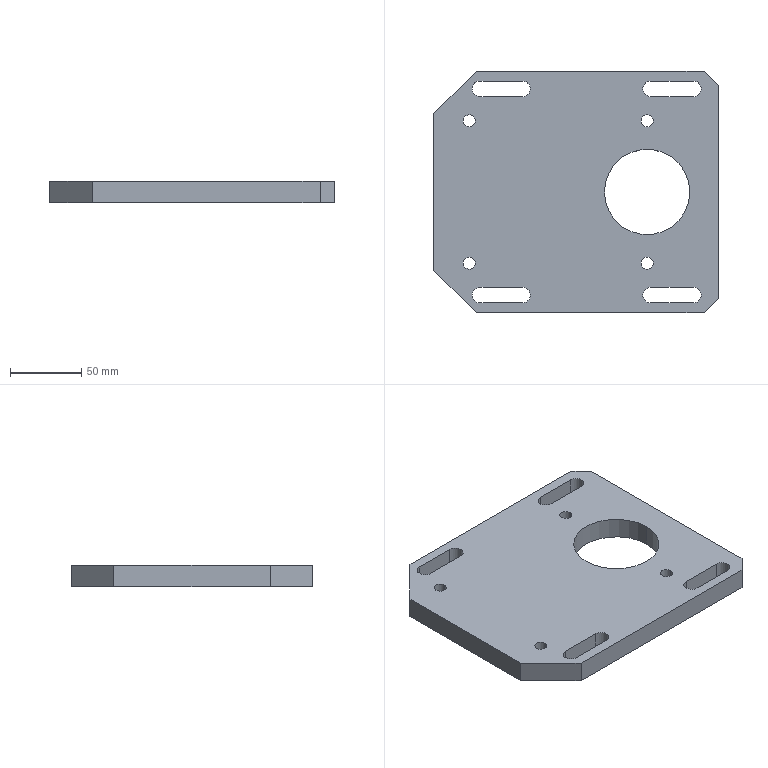CAM job | Mastercam | mm | 8 operations | part box 200 x 170 x 15
1. Contour (Ramp) | 1 - 8 平铣刀
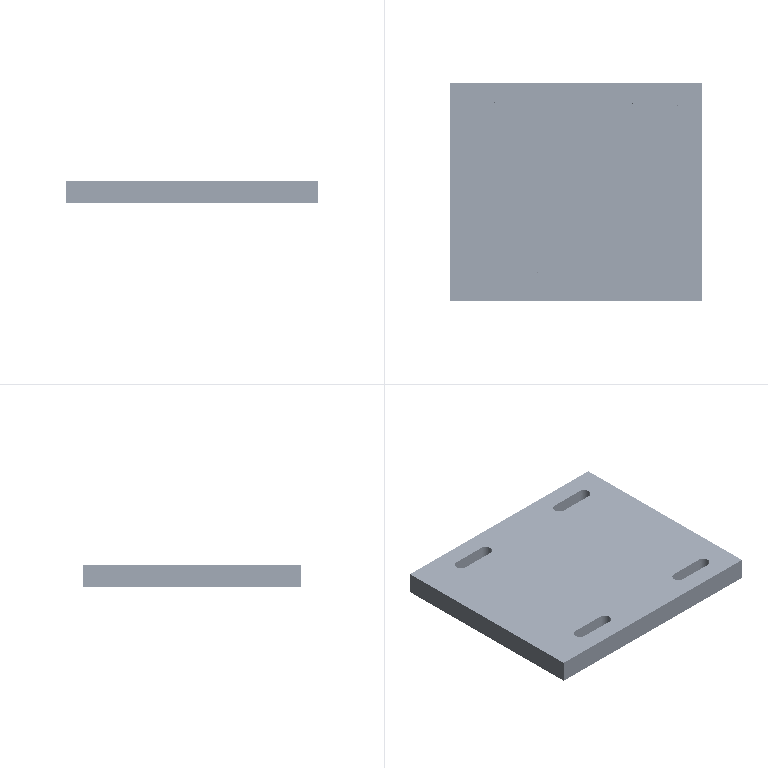2. 3D High Speed (Waterline) | 1 - 8 平铣刀
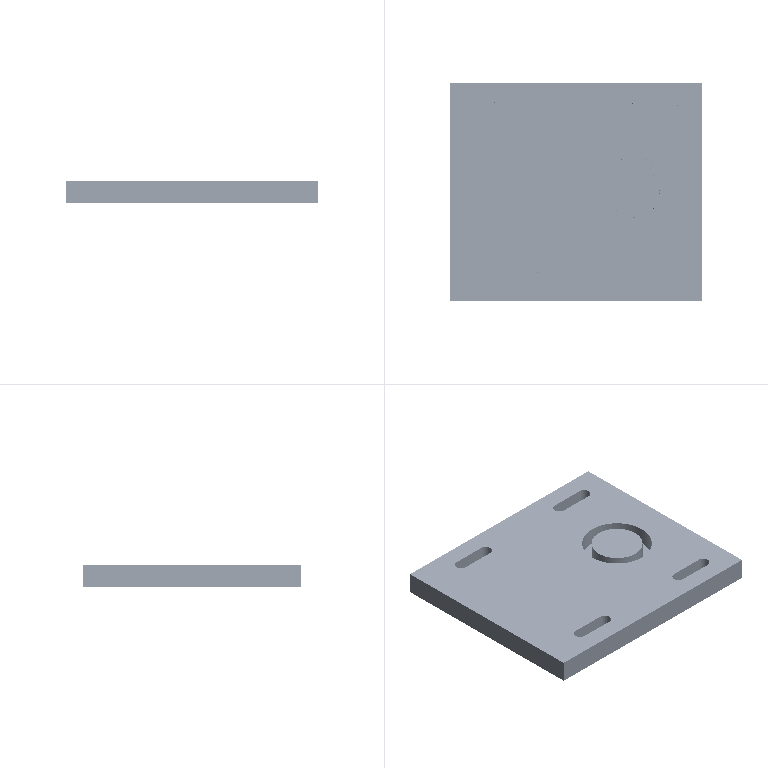3. Contour (Ramp) | 1 - 8 平铣刀
4. Contour (2D) | 2 - 8 平铣刀
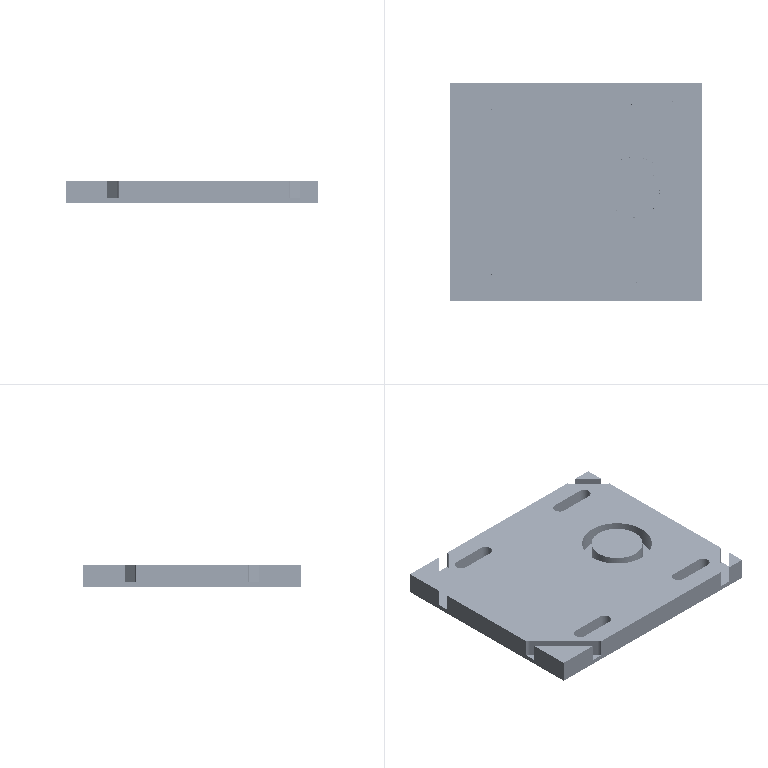5. Contour (2D) | 2 - 8 平铣刀
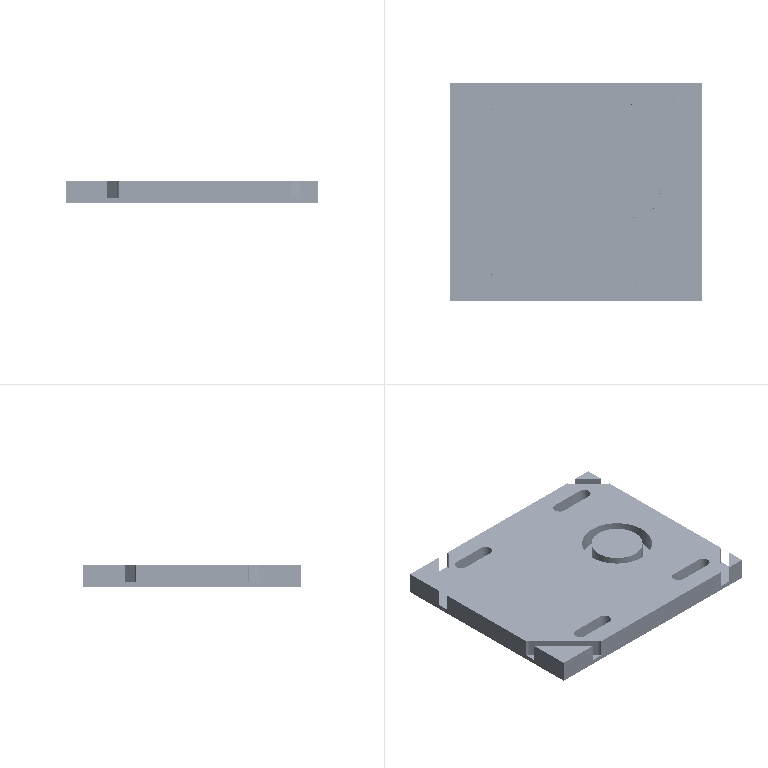6. Contour (2D) | 2 - 8 平铣刀
7. Drill/Counterbore | 3 - 6 倒角刀
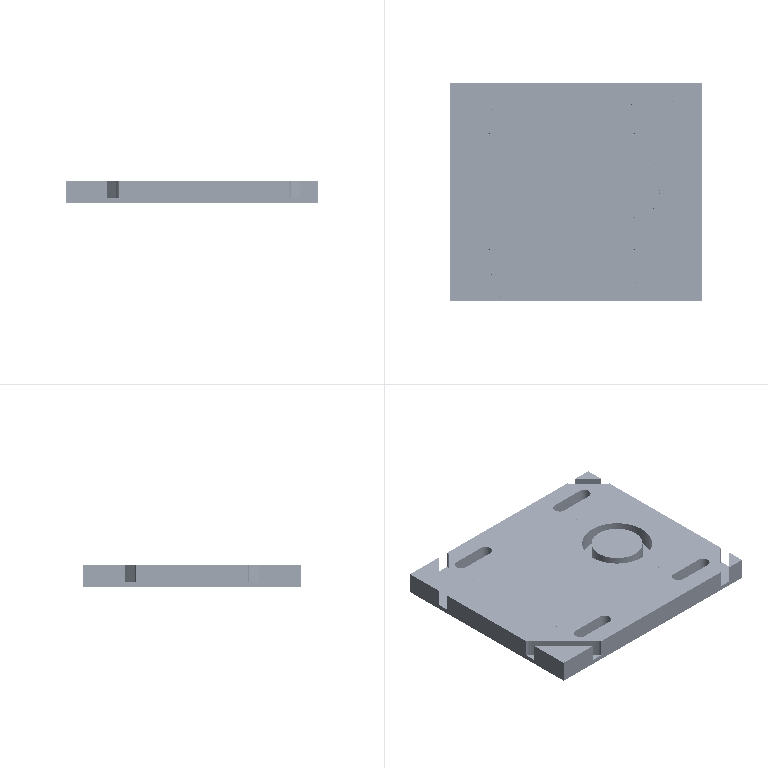8. Model Chamfer | 3 - 6 倒角刀